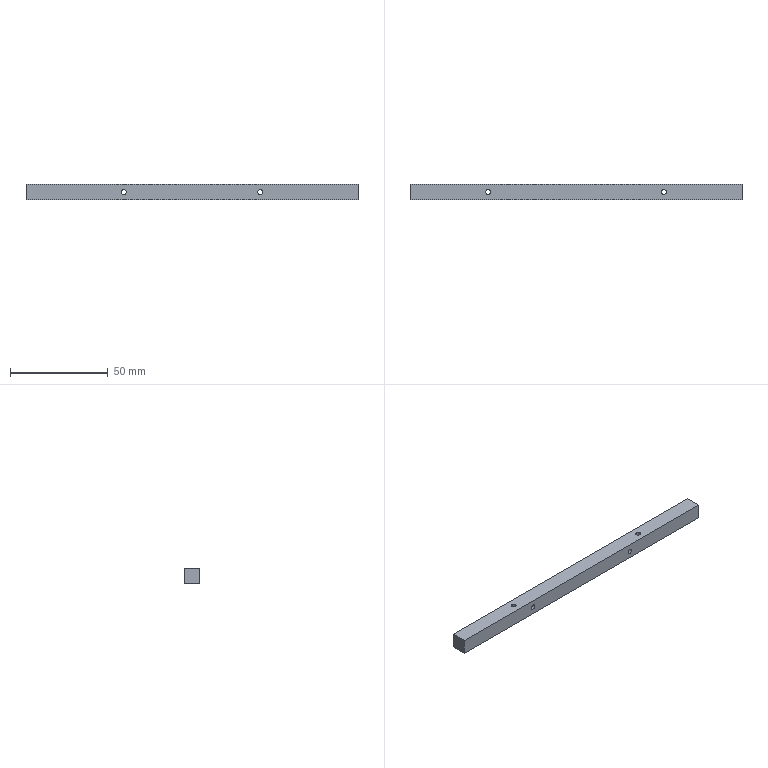CAM job | Mastercam | mm | 8 operations | part box 170 x 8 x 8
1. Facing | 24 - 100 平铣刀
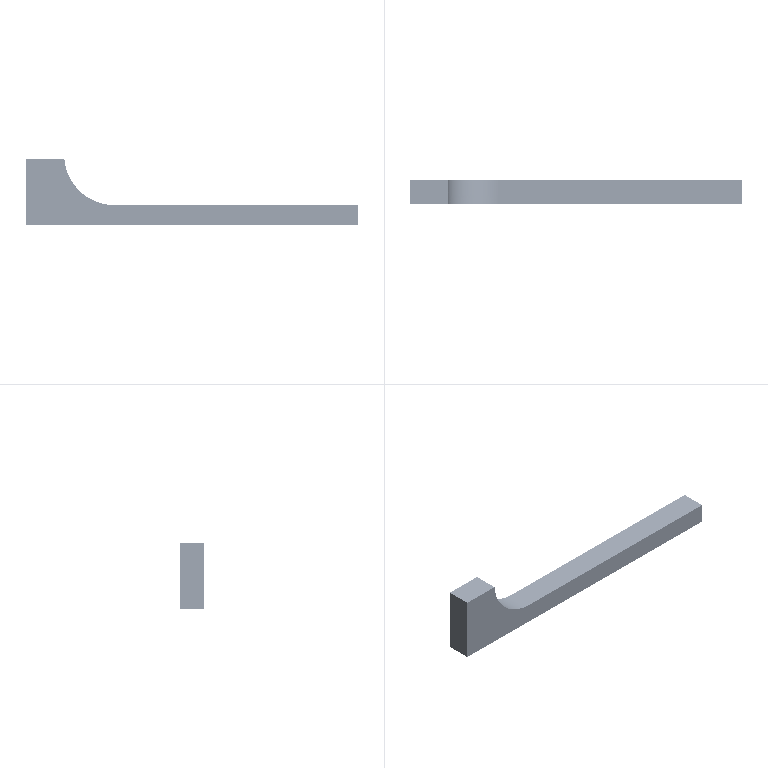2. Contour (Ramp) | 10 - 10 平铣刀
3. Contour (2D) | 10 - 10 平铣刀
4. Drill/Counterbore | 7 - 4 倒角刀
5. Contour (2D chamfer) | 7 - 4 倒角刀
6. Facing | 24 - 100 平铣刀
7. Contour (2D chamfer) | 7 - 4 倒角刀
8. Drill/Counterbore | 7 - 4 倒角刀